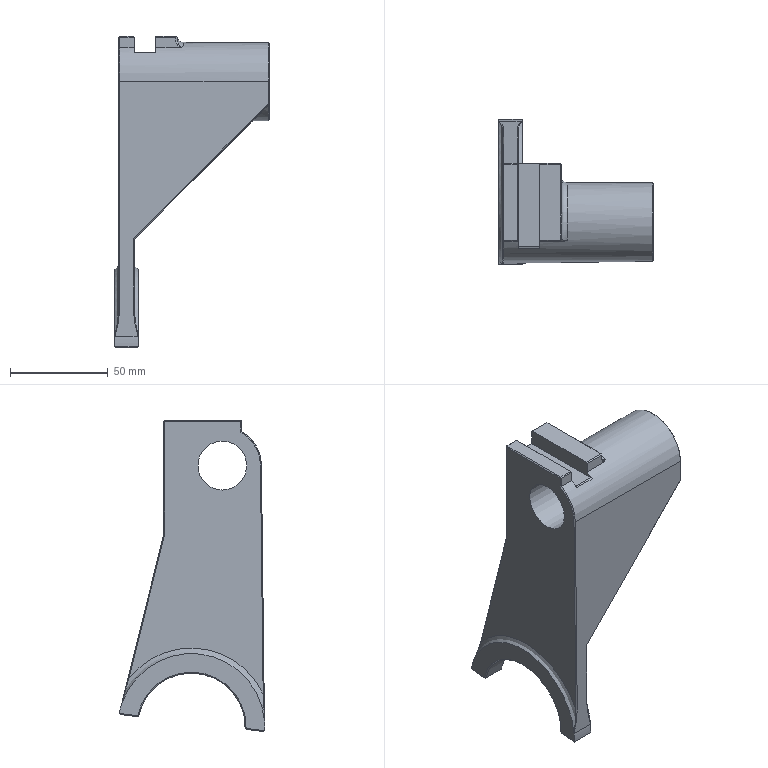Component | NX | BOCHALINGJIAN | 1 solid | 84 faces | volume 139398 mm3 | plane 58 | spline 10 | cylinder 8 | cone 5 | torus 3 | commonest cylinder face diameters 6 x3 75 x2 40 x1 25 x1 55 x1